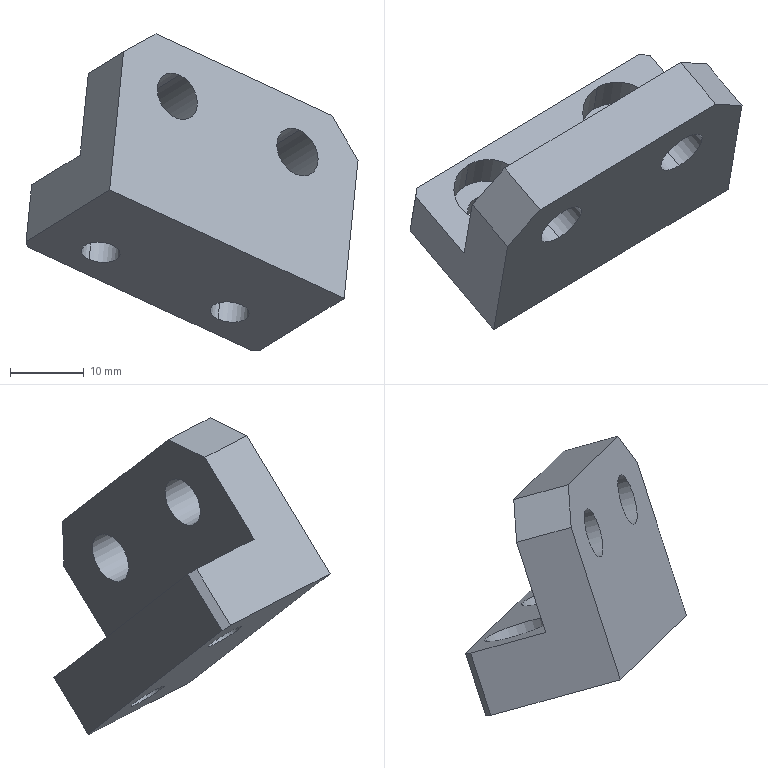Component | SolidWorks | 14AC-24-1-009-2 | 1 solid | 26 faces | box 45.12 x 37.53 x 42.96 mm | volume 11112 mm3 | plane 14 | cylinder 12 | commonest cylinder face diameters 10 x4 5.3 x4 6.8 x2 7 x2
build123d program:
from build123d import *

# Parameters (mm, degrees)
SKETCH1_W                                            = 27
SKETCH1_H                                            = 40
BOSS_EXTRUDE1_DEPTH                                  = 8
M8X1_0_TAPPED_HOLE1_D                                = 7
M8X1_0_TAPPED_HOLE1_DEPTH                            = 19
M8X1_0_TAPPED_HOLE1_TIP                              = 2.103
M8_TAPPED_HOLE1_D                                    = 6.8
M8_TAPPED_HOLE1_DEPTH                                = 19.75
M8_TAPPED_HOLE1_TIP                                  = 2.043
SKETCH6_W                                            = 9
SKETCH6_H                                            = 40
BOSS_EXTRUDE2_DEPTH                                  = 12
HOLE_SIZE_ACCORDING_TO_THE_TYPE_1_OF_HEX_D           = 5.3
HOLE_SIZE_ACCORDING_TO_THE_TYPE_1_OF_HEX_CBORE_D     = 10
HOLE_SIZE_ACCORDING_TO_THE_TYPE_1_OF_HEX_CBORE_DEPTH = 5.7
CHAMFER1_SIZE                                        = 5
CHAMFER2_SIZE                                        = 1


with BuildPart() as part:
    # Sketch1 → Boss-Extrude1 (new body)
    with BuildSketch(Plane.XY):
        Rectangle(SKETCH1_W, SKETCH1_H)
    extrude(amount=BOSS_EXTRUDE1_DEPTH)

    # M8x1.0 Tapped Hole1
    with Locations(Plane(origin=(5.5, 10, 8), x_dir=(1, 0, 0), z_dir=(0, 0, 1))):
        with Locations((0, 0)):
            Hole(M8X1_0_TAPPED_HOLE1_D / 2, depth=M8X1_0_TAPPED_HOLE1_DEPTH)
            with Locations((0, 0, -(M8X1_0_TAPPED_HOLE1_DEPTH + M8X1_0_TAPPED_HOLE1_TIP / 2))):  # 118° drill point
                Cone(0, M8X1_0_TAPPED_HOLE1_D / 2, M8X1_0_TAPPED_HOLE1_TIP, mode=Mode.SUBTRACT)

    # M8 Tapped Hole1
    with Locations(Plane(origin=(5.5, -10.5, 8), x_dir=(1, 0, 0), z_dir=(0, 0, 1))):
        with Locations((0, 0)):
            Hole(M8_TAPPED_HOLE1_D / 2, depth=M8_TAPPED_HOLE1_DEPTH)
            with Locations((0, 0, -(M8_TAPPED_HOLE1_DEPTH + M8_TAPPED_HOLE1_TIP / 2))):  # 118° drill point
                Cone(0, M8_TAPPED_HOLE1_D / 2, M8_TAPPED_HOLE1_TIP, mode=Mode.SUBTRACT)

    # Sketch6 → Boss-Extrude2 (add)
    with BuildSketch(Plane.XY.offset(8)):
        with Locations((-9, 0)):
            Rectangle(SKETCH6_W, SKETCH6_H)
    extrude(amount=BOSS_EXTRUDE2_DEPTH)

    # Hole Size according to the type 1 of hex (through all)
    with Locations(Plane(origin=(-4.5, 11, 14), x_dir=(0, 1, 0), z_dir=(1, 0, 0))):
        with Locations((0, 0), (-22, 0)):
            CounterBoreHole(HOLE_SIZE_ACCORDING_TO_THE_TYPE_1_OF_HEX_D / 2, HOLE_SIZE_ACCORDING_TO_THE_TYPE_1_OF_HEX_CBORE_D / 2, HOLE_SIZE_ACCORDING_TO_THE_TYPE_1_OF_HEX_CBORE_DEPTH)

    # Chamfer1
    chamfer1_edges = [part.edges().sort_by_distance(p)[0] for p in [
        (13.5, -20, 4),
        (13.5, 20, 4),
    ]]
    chamfer(chamfer1_edges, length=CHAMFER1_SIZE)

    # Chamfer2
    chamfer2_edges = [part.edges().sort_by_distance(p)[0] for p in [
        (-9, 20, 20),
        (-9, -20, 20),
    ]]
    chamfer(chamfer2_edges, length=CHAMFER2_SIZE)


solid = part.part

# Placed as in the assembly
solid = solid.moved(Location((533.188, -316.638, -28.905), (-117.442, -36.759, -83.855)))
STEP:
#1=COLOUR_RGB('',0.7922,0.8196,0.9333);
#2=FILL_AREA_STYLE_COLOUR('',#1);
#3=FILL_AREA_STYLE('',(#2));
#4=SURFACE_STYLE_FILL_AREA(#3);
#5=SURFACE_SIDE_STYLE('',(#4));
#6=SURFACE_STYLE_USAGE(.BOTH.,#5);
#7=PRESENTATION_STYLE_ASSIGNMENT((#6));
#8=CARTESIAN_POINT('',(20.855,-11.934,-1.917));
#9=VERTEX_POINT('',#8);
#10=CARTESIAN_POINT('',(21.09,-12.214,-1.771));
#11=VERTEX_POINT('',#10);
#12=CARTESIAN_POINT('',(20.972,-12.074,-1.844));
#13=DIRECTION('',(0.08576,0.5151,0.8529));
#14=DIRECTION('',(0.5985,-0.711,0.3692));
#15=AXIS2_PLACEMENT_3D('',#12,#13,#14);
#16=CIRCLE('',#15,0.1969);
#17=EDGE_CURVE('',#9,#11,#16,.T.);
#18=ORIENTED_EDGE('',*,*,#17,.F.);
#19=CARTESIAN_POINT('',(20.874,-11.818,-1.725));
#20=VERTEX_POINT('',#19);
#21=CARTESIAN_POINT('',(20.874,-11.818,-1.725));
#22=DIRECTION('',(0.08576,0.5151,0.8529));
#23=VECTOR('',#22,39.37);
#24=LINE('',#21,#23);
#25=EDGE_CURVE('',#9,#20,#24,.T.);
#26=ORIENTED_EDGE('',*,*,#25,.T.);
#27=CARTESIAN_POINT('',(21.109,-12.098,-1.58));
#28=VERTEX_POINT('',#27);
#29=CARTESIAN_POINT('',(20.992,-11.958,-1.652));
#30=DIRECTION('',(0.08576,0.5151,0.8529));
#31=DIRECTION('',(0.5985,-0.711,0.3692));
#32=AXIS2_PLACEMENT_3D('',#29,#30,#31);
#33=CIRCLE('',#32,0.1969);
#34=EDGE_CURVE('',#20,#28,#33,.T.);
#35=ORIENTED_EDGE('',*,*,#34,.T.);
#36=CARTESIAN_POINT('',(21.109,-12.098,-1.58));
#37=DIRECTION('',(0.08576,0.5151,0.8529));
#38=VECTOR('',#37,39.37);
#39=LINE('',#36,#38);
#40=EDGE_CURVE('',#11,#28,#39,.T.);
#41=ORIENTED_EDGE('',*,*,#40,.F.);
#42=EDGE_LOOP('',(#18,#26,#35,#41));
#43=FACE_OUTER_BOUND('',#42,.T.);
#44=CARTESIAN_POINT('',(20.992,-11.958,-1.652));
#45=DIRECTION('',(0.08576,0.5151,0.8529));
#46=DIRECTION('',(0.5985,-0.711,0.3692));
#47=AXIS2_PLACEMENT_3D('',#44,#45,#46);
#48=CYLINDRICAL_SURFACE('',#47,0.1969);
#49=ADVANCED_FACE('',(#43),#48,.F.);
#50=CARTESIAN_POINT('',(20.899,-12.066,-1.993));
#51=VERTEX_POINT('',#50);
#52=CARTESIAN_POINT('',(21.024,-12.215,-1.916));
#53=VERTEX_POINT('',#52);
#54=CARTESIAN_POINT('',(20.961,-12.141,-1.955));
#55=DIRECTION('',(0.08576,0.5151,0.8529));
#56=DIRECTION('',(0.5985,-0.711,0.3692));
#57=AXIS2_PLACEMENT_3D('',#54,#55,#56);
#58=CIRCLE('',#57,0.1043);
#59=EDGE_CURVE('',#51,#53,#58,.T.);
#60=ORIENTED_EDGE('',*,*,#59,.F.);
#61=CARTESIAN_POINT('',(20.91,-11.999,-1.882));
#62=VERTEX_POINT('',#61);
#63=CARTESIAN_POINT('',(20.929,-11.884,-1.691));
#64=DIRECTION('',(0.08576,0.5151,0.8529));
#65=VECTOR('',#64,39.37);
#66=LINE('',#63,#65);
#67=EDGE_CURVE('',#51,#62,#66,.T.);
#68=ORIENTED_EDGE('',*,*,#67,.T.);
#69=CARTESIAN_POINT('',(21.035,-12.148,-1.805));
#70=VERTEX_POINT('',#69);
#71=CARTESIAN_POINT('',(20.972,-12.074,-1.844));
#72=DIRECTION('',(0.08576,0.5151,0.8529));
#73=DIRECTION('',(0.5985,-0.711,0.3692));
#74=AXIS2_PLACEMENT_3D('',#71,#72,#73);
#75=CIRCLE('',#74,0.1043);
#76=EDGE_CURVE('',#62,#70,#75,.T.);
#77=ORIENTED_EDGE('',*,*,#76,.T.);
#78=CARTESIAN_POINT('',(21.054,-12.032,-1.614));
#79=DIRECTION('',(0.08576,0.5151,0.8529));
#80=VECTOR('',#79,39.37);
#81=LINE('',#78,#80);
#82=EDGE_CURVE('',#53,#70,#81,.T.);
#83=ORIENTED_EDGE('',*,*,#82,.F.);
#84=EDGE_LOOP('',(#60,#68,#77,#83));
#85=FACE_OUTER_BOUND('',#84,.T.);
#86=CARTESIAN_POINT('',(20.992,-11.958,-1.652));
#87=DIRECTION('',(0.08576,0.5151,0.8529));
#88=DIRECTION('',(0.5985,-0.711,0.3692));
#89=AXIS2_PLACEMENT_3D('',#86,#87,#88);
#90=CYLINDRICAL_SURFACE('',#89,0.1043);
#91=ADVANCED_FACE('',(#85),#90,.F.);
#92=CARTESIAN_POINT('',(20.165,-12.348,-1.597));
#93=VERTEX_POINT('',#92);
#94=CARTESIAN_POINT('',(20.4,-12.628,-1.451));
#95=VERTEX_POINT('',#94);
#96=CARTESIAN_POINT('',(20.282,-12.488,-1.524));
#97=DIRECTION('',(0.08576,0.5151,0.8529));
#98=DIRECTION('',(0.5985,-0.711,0.3692));
#99=AXIS2_PLACEMENT_3D('',#96,#97,#98);
#100=CIRCLE('',#99,0.1969);
#101=EDGE_CURVE('',#93,#95,#100,.T.);
#102=ORIENTED_EDGE('',*,*,#101,.F.);
#103=CARTESIAN_POINT('',(20.184,-12.233,-1.405));
#104=VERTEX_POINT('',#103);
#105=CARTESIAN_POINT('',(20.184,-12.233,-1.405));
#106=DIRECTION('',(0.08576,0.5151,0.8529));
#107=VECTOR('',#106,39.37);
#108=LINE('',#105,#107);
#109=EDGE_CURVE('',#93,#104,#108,.T.);
#110=ORIENTED_EDGE('',*,*,#109,.T.);
#111=CARTESIAN_POINT('',(20.419,-12.513,-1.26));
#112=VERTEX_POINT('',#111);
#113=CARTESIAN_POINT('',(20.302,-12.373,-1.333));
#114=DIRECTION('',(0.08576,0.5151,0.8529));
#115=DIRECTION('',(0.5985,-0.711,0.3692));
#116=AXIS2_PLACEMENT_3D('',#113,#114,#115);
#117=CIRCLE('',#116,0.1969);
#118=EDGE_CURVE('',#104,#112,#117,.T.);
#119=ORIENTED_EDGE('',*,*,#118,.T.);
#120=CARTESIAN_POINT('',(20.419,-12.513,-1.26));
#121=DIRECTION('',(0.08576,0.5151,0.8529));
#122=VECTOR('',#121,39.37);
#123=LINE('',#120,#122);
#124=EDGE_CURVE('',#95,#112,#123,.T.);
#125=ORIENTED_EDGE('',*,*,#124,.F.);
#126=EDGE_LOOP('',(#102,#110,#119,#125));
#127=FACE_OUTER_BOUND('',#126,.T.);
#128=CARTESIAN_POINT('',(20.302,-12.373,-1.333));
#129=DIRECTION('',(0.08576,0.5151,0.8529));
#130=DIRECTION('',(0.5985,-0.711,0.3692));
#131=AXIS2_PLACEMENT_3D('',#128,#129,#130);
#132=CYLINDRICAL_SURFACE('',#131,0.1969);
#133=ADVANCED_FACE('',(#127),#132,.F.);
#134=CARTESIAN_POINT('',(20.209,-12.481,-1.673));
#135=VERTEX_POINT('',#134);
#136=CARTESIAN_POINT('',(20.334,-12.629,-1.596));
#137=VERTEX_POINT('',#136);
#138=CARTESIAN_POINT('',(20.271,-12.555,-1.635));
#139=DIRECTION('',(0.08576,0.5151,0.8529));
#140=DIRECTION('',(0.5985,-0.711,0.3692));
#141=AXIS2_PLACEMENT_3D('',#138,#139,#140);
#142=CIRCLE('',#141,0.1043);
#143=EDGE_CURVE('',#135,#137,#142,.T.);
#144=ORIENTED_EDGE('',*,*,#143,.F.);
#145=CARTESIAN_POINT('',(20.22,-12.414,-1.563));
#146=VERTEX_POINT('',#145);
#147=CARTESIAN_POINT('',(20.239,-12.299,-1.371));
#148=DIRECTION('',(0.08576,0.5151,0.8529));
#149=VECTOR('',#148,39.37);
#150=LINE('',#147,#149);
#151=EDGE_CURVE('',#135,#146,#150,.T.);
#152=ORIENTED_EDGE('',*,*,#151,.T.);
#153=CARTESIAN_POINT('',(20.345,-12.562,-1.486));
#154=VERTEX_POINT('',#153);
#155=CARTESIAN_POINT('',(20.282,-12.488,-1.524));
#156=DIRECTION('',(0.08576,0.5151,0.8529));
#157=DIRECTION('',(0.5985,-0.711,0.3692));
#158=AXIS2_PLACEMENT_3D('',#155,#156,#157);
#159=CIRCLE('',#158,0.1043);
#160=EDGE_CURVE('',#146,#154,#159,.T.);
#161=ORIENTED_EDGE('',*,*,#160,.T.);
#162=CARTESIAN_POINT('',(20.364,-12.447,-1.294));
#163=DIRECTION('',(0.08576,0.5151,0.8529));
#164=VECTOR('',#163,39.37);
#165=LINE('',#162,#164);
#166=EDGE_CURVE('',#137,#154,#165,.T.);
#167=ORIENTED_EDGE('',*,*,#166,.F.);
#168=EDGE_LOOP('',(#144,#152,#161,#167));
#169=FACE_OUTER_BOUND('',#168,.T.);
#170=CARTESIAN_POINT('',(20.302,-12.373,-1.333));
#171=DIRECTION('',(0.08576,0.5151,0.8529));
#172=DIRECTION('',(0.5985,-0.711,0.3692));
#173=AXIS2_PLACEMENT_3D('',#170,#171,#172);
#174=CYLINDRICAL_SURFACE('',#173,0.1043);
#175=ADVANCED_FACE('',(#169),#174,.F.);
#176=CARTESIAN_POINT('',(20.669,-12.621,-0.9148));
#177=VERTEX_POINT('',#176);
#178=CARTESIAN_POINT('',(20.692,-12.483,-0.6865));
#179=VERTEX_POINT('',#178);
#180=CARTESIAN_POINT('',(20.681,-12.552,-0.8007));
#181=DIRECTION('',(-0.5985,0.711,-0.3692));
#182=DIRECTION('',(0.08576,0.5151,0.8529));
#183=AXIS2_PLACEMENT_3D('',#180,#181,#182);
#184=CIRCLE('',#183,0.1339);
#185=EDGE_CURVE('',#177,#179,#184,.T.);
#186=ORIENTED_EDGE('',*,*,#185,.F.);
#187=CARTESIAN_POINT('',(20.481,-12.397,-1.031));
#188=VERTEX_POINT('',#187);
#189=CARTESIAN_POINT('',(20.481,-12.397,-1.031));
#190=DIRECTION('',(-0.5985,0.711,-0.3692));
#191=VECTOR('',#190,39.37);
#192=LINE('',#189,#191);
#193=EDGE_CURVE('',#177,#188,#192,.T.);
#194=ORIENTED_EDGE('',*,*,#193,.T.);
#195=CARTESIAN_POINT('',(20.504,-12.26,-0.8028));
#196=VERTEX_POINT('',#195);
#197=CARTESIAN_POINT('',(20.492,-12.328,-0.917));
#198=DIRECTION('',(-0.5985,0.711,-0.3692));
#199=DIRECTION('',(0.08576,0.5151,0.8529));
#200=AXIS2_PLACEMENT_3D('',#197,#198,#199);
#201=CIRCLE('',#200,0.1339);
#202=EDGE_CURVE('',#188,#196,#201,.T.);
#203=ORIENTED_EDGE('',*,*,#202,.T.);
#204=CARTESIAN_POINT('',(20.504,-12.26,-0.8028));
#205=DIRECTION('',(-0.5985,0.711,-0.3692));
#206=VECTOR('',#205,39.37);
#207=LINE('',#204,#206);
#208=EDGE_CURVE('',#179,#196,#207,.T.);
#209=ORIENTED_EDGE('',*,*,#208,.F.);
#210=EDGE_LOOP('',(#186,#194,#203,#209));
#211=FACE_OUTER_BOUND('',#210,.T.);
#212=CARTESIAN_POINT('',(20.492,-12.328,-0.917));
#213=DIRECTION('',(-0.5985,0.711,-0.3692));
#214=DIRECTION('',(0.08576,0.5151,0.8529));
#215=AXIS2_PLACEMENT_3D('',#212,#213,#214);
#216=CYLINDRICAL_SURFACE('',#215,0.1339);
#217=ADVANCED_FACE('',(#211),#216,.F.);
#218=CARTESIAN_POINT('',(21.312,-12.237,-1.216));
#219=VERTEX_POINT('',#218);
#220=CARTESIAN_POINT('',(21.336,-12.095,-0.9811));
#221=VERTEX_POINT('',#220);
#222=CARTESIAN_POINT('',(21.324,-12.166,-1.099));
#223=DIRECTION('',(-0.5985,0.711,-0.3692));
#224=DIRECTION('',(0.08576,0.5151,0.8529));
#225=AXIS2_PLACEMENT_3D('',#222,#223,#224);
#226=CIRCLE('',#225,0.1378);
#227=EDGE_CURVE('',#219,#221,#226,.T.);
#228=ORIENTED_EDGE('',*,*,#227,.F.);
#229=CARTESIAN_POINT('',(21.124,-12.013,-1.332));
#230=VERTEX_POINT('',#229);
#231=CARTESIAN_POINT('',(21.124,-12.013,-1.332));
#232=DIRECTION('',(-0.5985,0.711,-0.3692));
#233=VECTOR('',#232,39.37);
#234=LINE('',#231,#233);
#235=EDGE_CURVE('',#219,#230,#234,.T.);
#236=ORIENTED_EDGE('',*,*,#235,.T.);
#237=CARTESIAN_POINT('',(21.147,-11.871,-1.097));
#238=VERTEX_POINT('',#237);
#239=CARTESIAN_POINT('',(21.135,-11.942,-1.215));
#240=DIRECTION('',(-0.5985,0.711,-0.3692));
#241=DIRECTION('',(0.08576,0.5151,0.8529));
#242=AXIS2_PLACEMENT_3D('',#239,#240,#241);
#243=CIRCLE('',#242,0.1378);
#244=EDGE_CURVE('',#230,#238,#243,.T.);
#245=ORIENTED_EDGE('',*,*,#244,.T.);
#246=CARTESIAN_POINT('',(21.147,-11.871,-1.097));
#247=DIRECTION('',(-0.5985,0.711,-0.3692));
#248=VECTOR('',#247,39.37);
#249=LINE('',#246,#248);
#250=EDGE_CURVE('',#221,#238,#249,.T.);
#251=ORIENTED_EDGE('',*,*,#250,.F.);
#252=EDGE_LOOP('',(#228,#236,#245,#251));
#253=FACE_OUTER_BOUND('',#252,.T.);
#254=CARTESIAN_POINT('',(21.135,-11.942,-1.215));
#255=DIRECTION('',(-0.5985,0.711,-0.3692));
#256=DIRECTION('',(0.08576,0.5151,0.8529));
#257=AXIS2_PLACEMENT_3D('',#254,#255,#256);
#258=CYLINDRICAL_SURFACE('',#257,0.1378);
#259=ADVANCED_FACE('',(#253),#258,.F.);
#260=CARTESIAN_POINT('',(20.378,-12.251,-0.5829));
#261=VERTEX_POINT('',#260);
#262=CARTESIAN_POINT('',(21.319,-11.686,-1.019));
#263=VERTEX_POINT('',#262);
#264=CARTESIAN_POINT('',(21.476,-11.591,-1.092));
#265=DIRECTION('',(0.7966,0.4787,-0.3692));
#266=VECTOR('',#265,39.37);
#267=LINE('',#264,#266);
#268=EDGE_CURVE('',#261,#263,#267,.T.);
#269=ORIENTED_EDGE('',*,*,#268,.F.);
#270=CARTESIAN_POINT('',(20.567,-12.475,-0.4666));
#271=VERTEX_POINT('',#270);
#272=CARTESIAN_POINT('',(20.378,-12.251,-0.5829));
#273=DIRECTION('',(0.5985,-0.711,0.3692));
#274=VECTOR('',#273,39.37);
#275=LINE('',#272,#274);
#276=EDGE_CURVE('',#261,#271,#275,.T.);
#277=ORIENTED_EDGE('',*,*,#276,.T.);
#278=CARTESIAN_POINT('',(21.508,-11.91,-0.9027));
#279=VERTEX_POINT('',#278);
#280=CARTESIAN_POINT('',(21.664,-11.815,-0.9754));
#281=DIRECTION('',(0.7966,0.4787,-0.3692));
#282=VECTOR('',#281,39.37);
#283=LINE('',#280,#282);
#284=EDGE_CURVE('',#271,#279,#283,.T.);
#285=ORIENTED_EDGE('',*,*,#284,.T.);
#286=CARTESIAN_POINT('',(21.319,-11.686,-1.019));
#287=DIRECTION('',(-0.5985,0.711,-0.3692));
#288=VECTOR('',#287,39.37);
#289=LINE('',#286,#288);
#290=EDGE_CURVE('',#279,#263,#289,.T.);
#291=ORIENTED_EDGE('',*,*,#290,.T.);
#292=EDGE_LOOP('',(#269,#277,#285,#291));
#293=FACE_OUTER_BOUND('',#292,.T.);
#294=CARTESIAN_POINT('',(21.476,-11.591,-1.092));
#295=DIRECTION('',(-0.08576,-0.5151,-0.8529));
#296=DIRECTION('',(-0.7966,-0.4787,0.3692));
#297=AXIS2_PLACEMENT_3D('',#294,#295,#296);
#298=PLANE('',#297);
#299=ADVANCED_FACE('',(#293),#298,.F.);
#300=CARTESIAN_POINT('',(21.126,-11.831,-2.158));
#301=VERTEX_POINT('',#300);
#302=CARTESIAN_POINT('',(21.573,-12.363,-1.882));
#303=VERTEX_POINT('',#302);
#304=CARTESIAN_POINT('',(21.385,-12.139,-1.998));
#305=DIRECTION('',(0.5985,-0.711,0.3692));
#306=VECTOR('',#305,39.37);
#307=LINE('',#304,#306);
#308=EDGE_CURVE('',#301,#303,#307,.T.);
#309=ORIENTED_EDGE('',*,*,#308,.F.);
#310=CARTESIAN_POINT('',(21.156,-11.648,-1.856));
#311=VERTEX_POINT('',#310);
#312=CARTESIAN_POINT('',(21.156,-11.648,-1.856));
#313=DIRECTION('',(0.08576,0.5151,0.8529));
#314=VECTOR('',#313,39.37);
#315=LINE('',#312,#314);
#316=EDGE_CURVE('',#301,#311,#315,.T.);
#317=ORIENTED_EDGE('',*,*,#316,.T.);
#318=CARTESIAN_POINT('',(21.415,-11.956,-1.696));
#319=VERTEX_POINT('',#318);
#320=CARTESIAN_POINT('',(21.132,-11.621,-1.871));
#321=DIRECTION('',(0.5985,-0.711,0.3692));
#322=VECTOR('',#321,39.37);
#323=LINE('',#320,#322);
#324=EDGE_CURVE('',#311,#319,#323,.T.);
#325=ORIENTED_EDGE('',*,*,#324,.T.);
#326=CARTESIAN_POINT('',(21.459,-11.693,-1.26));
#327=VERTEX_POINT('',#326);
#328=CARTESIAN_POINT('',(21.385,-12.139,-1.998));
#329=DIRECTION('',(-0.08576,-0.5151,-0.8529));
#330=VECTOR('',#329,39.37);
#331=LINE('',#328,#330);
#332=EDGE_CURVE('',#327,#319,#331,.T.);
#333=ORIENTED_EDGE('',*,*,#332,.F.);
#334=CARTESIAN_POINT('',(21.648,-11.917,-1.143));
#335=VERTEX_POINT('',#334);
#336=CARTESIAN_POINT('',(21.459,-11.693,-1.26));
#337=DIRECTION('',(0.5985,-0.711,0.3692));
#338=VECTOR('',#337,39.37);
#339=LINE('',#336,#338);
#340=EDGE_CURVE('',#327,#335,#339,.T.);
#341=ORIENTED_EDGE('',*,*,#340,.T.);
#342=CARTESIAN_POINT('',(21.573,-12.363,-1.882));
#343=DIRECTION('',(-0.08576,-0.5151,-0.8529));
#344=VECTOR('',#343,39.37);
#345=LINE('',#342,#344);
#346=EDGE_CURVE('',#335,#303,#345,.T.);
#347=ORIENTED_EDGE('',*,*,#346,.T.);
#348=EDGE_LOOP('',(#309,#317,#325,#333,#341,#347));
#349=FACE_OUTER_BOUND('',#348,.T.);
#350=CARTESIAN_POINT('',(21.385,-12.139,-1.998));
#351=DIRECTION('',(-0.7966,-0.4787,0.3692));
#352=DIRECTION('',(0.5985,-0.711,0.3692));
#353=AXIS2_PLACEMENT_3D('',#350,#351,#352);
#354=PLANE('',#353);
#355=ADVANCED_FACE('',(#349),#354,.F.);
#356=CARTESIAN_POINT('',(20.961,-12.141,-1.955));
#357=DIRECTION('',(0.08576,0.5151,0.8529));
#358=DIRECTION('',(0.5985,-0.711,0.3692));
#359=AXIS2_PLACEMENT_3D('',#356,#357,#358);
#360=CIRCLE('',#359,0.1043);
#361=EDGE_CURVE('',#53,#51,#360,.T.);
#362=ORIENTED_EDGE('',*,*,#361,.T.);
#363=ORIENTED_EDGE('',*,*,#59,.T.);
#364=EDGE_LOOP('',(#362,#363));
#365=FACE_BOUND('',#364,.T.);
#366=CARTESIAN_POINT('',(20.271,-12.555,-1.635));
#367=DIRECTION('',(0.08576,0.5151,0.8529));
#368=DIRECTION('',(0.5985,-0.711,0.3692));
#369=AXIS2_PLACEMENT_3D('',#366,#367,#368);
#370=CIRCLE('',#369,0.1043);
#371=EDGE_CURVE('',#137,#135,#370,.T.);
#372=ORIENTED_EDGE('',*,*,#371,.T.);
#373=ORIENTED_EDGE('',*,*,#143,.T.);
#374=EDGE_LOOP('',(#372,#373));
#375=FACE_BOUND('',#374,.T.);
#376=CARTESIAN_POINT('',(21.071,-11.822,-2.158));
#377=VERTEX_POINT('',#376);
#378=CARTESIAN_POINT('',(19.879,-12.538,-1.606));
#379=VERTEX_POINT('',#378);
#380=CARTESIAN_POINT('',(21.102,-11.803,-2.173));
#381=DIRECTION('',(-0.7966,-0.4787,0.3692));
#382=VECTOR('',#381,39.37);
#383=LINE('',#380,#382);
#384=EDGE_CURVE('',#377,#379,#383,.T.);
#385=ORIENTED_EDGE('',*,*,#384,.F.);
#386=CARTESIAN_POINT('',(21.071,-11.822,-2.158));
#387=DIRECTION('',(0.9864,-0.1642,0.));
#388=VECTOR('',#387,39.37);
#389=LINE('',#386,#388);
#390=EDGE_CURVE('',#377,#301,#389,.T.);
#391=ORIENTED_EDGE('',*,*,#390,.T.);
#392=ORIENTED_EDGE('',*,*,#308,.T.);
#393=CARTESIAN_POINT('',(20.319,-13.117,-1.301));
#394=VERTEX_POINT('',#393);
#395=CARTESIAN_POINT('',(21.573,-12.363,-1.882));
#396=DIRECTION('',(-0.7966,-0.4787,0.3692));
#397=VECTOR('',#396,39.37);
#398=LINE('',#395,#397);
#399=EDGE_CURVE('',#303,#394,#398,.T.);
#400=ORIENTED_EDGE('',*,*,#399,.T.);
#401=CARTESIAN_POINT('',(19.871,-12.585,-1.577));
#402=VERTEX_POINT('',#401);
#403=CARTESIAN_POINT('',(20.13,-12.893,-1.417));
#404=DIRECTION('',(0.5985,-0.711,0.3692));
#405=VECTOR('',#404,39.37);
#406=LINE('',#403,#405);
#407=EDGE_CURVE('',#402,#394,#406,.T.);
#408=ORIENTED_EDGE('',*,*,#407,.F.);
#409=CARTESIAN_POINT('',(19.879,-12.538,-1.606));
#410=DIRECTION('',(0.1401,0.8413,-0.5222));
#411=VECTOR('',#410,39.37);
#412=LINE('',#409,#411);
#413=EDGE_CURVE('',#402,#379,#412,.T.);
#414=ORIENTED_EDGE('',*,*,#413,.T.);
#415=EDGE_LOOP('',(#385,#391,#392,#400,#408,#414));
#416=FACE_OUTER_BOUND('',#415,.T.);
#417=CARTESIAN_POINT('',(21.385,-12.139,-1.998));
#418=DIRECTION('',(0.08576,0.5151,0.8529));
#419=DIRECTION('',(0.7966,0.4787,-0.3692));
#420=AXIS2_PLACEMENT_3D('',#417,#418,#419);
#421=PLANE('',#420);
#422=ADVANCED_FACE('',(#365,#375,#416),#421,.F.);
#423=CARTESIAN_POINT('',(19.902,-12.402,-1.275));
#424=VERTEX_POINT('',#423);
#425=CARTESIAN_POINT('',(20.161,-12.71,-1.115));
#426=VERTEX_POINT('',#425);
#427=CARTESIAN_POINT('',(19.878,-12.374,-1.289));
#428=DIRECTION('',(0.5985,-0.711,0.3692));
#429=VECTOR('',#428,39.37);
#430=LINE('',#427,#429);
#431=EDGE_CURVE('',#424,#426,#430,.T.);
#432=ORIENTED_EDGE('',*,*,#431,.F.);
#433=CARTESIAN_POINT('',(19.871,-12.585,-1.577));
#434=DIRECTION('',(-0.08576,-0.5151,-0.8529));
#435=VECTOR('',#434,39.37);
#436=LINE('',#433,#435);
#437=EDGE_CURVE('',#424,#402,#436,.T.);
#438=ORIENTED_EDGE('',*,*,#437,.T.);
#439=ORIENTED_EDGE('',*,*,#407,.T.);
#440=CARTESIAN_POINT('',(20.393,-12.671,-0.5618));
#441=VERTEX_POINT('',#440);
#442=CARTESIAN_POINT('',(20.319,-13.117,-1.301));
#443=DIRECTION('',(0.08576,0.5151,0.8529));
#444=VECTOR('',#443,39.37);
#445=LINE('',#442,#444);
#446=EDGE_CURVE('',#394,#441,#445,.T.);
#447=ORIENTED_EDGE('',*,*,#446,.T.);
#448=CARTESIAN_POINT('',(20.205,-12.447,-0.6781));
#449=VERTEX_POINT('',#448);
#450=CARTESIAN_POINT('',(20.205,-12.447,-0.6781));
#451=DIRECTION('',(-0.5985,0.711,-0.3692));
#452=VECTOR('',#451,39.37);
#453=LINE('',#450,#452);
#454=EDGE_CURVE('',#441,#449,#453,.T.);
#455=ORIENTED_EDGE('',*,*,#454,.T.);
#456=CARTESIAN_POINT('',(20.13,-12.893,-1.417));
#457=DIRECTION('',(0.08576,0.5151,0.8529));
#458=VECTOR('',#457,39.37);
#459=LINE('',#456,#458);
#460=EDGE_CURVE('',#426,#449,#459,.T.);
#461=ORIENTED_EDGE('',*,*,#460,.F.);
#462=EDGE_LOOP('',(#432,#438,#439,#447,#455,#461));
#463=FACE_OUTER_BOUND('',#462,.T.);
#464=CARTESIAN_POINT('',(20.13,-12.893,-1.417));
#465=DIRECTION('',(0.7966,0.4787,-0.3692));
#466=DIRECTION('',(-0.5985,0.711,-0.3692));
#467=AXIS2_PLACEMENT_3D('',#464,#465,#466);
#468=PLANE('',#467);
#469=ADVANCED_FACE('',(#463),#468,.F.);
#470=ORIENTED_EDGE('',*,*,#460,.T.);
#471=CARTESIAN_POINT('',(20.404,-12.222,-0.5687));
#472=DIRECTION('',(0.6239,0.7027,0.342));
#473=VECTOR('',#472,39.37);
#474=LINE('',#471,#473);
#475=EDGE_CURVE('',#449,#261,#474,.T.);
#476=ORIENTED_EDGE('',*,*,#475,.T.);
#477=ORIENTED_EDGE('',*,*,#268,.T.);
#478=CARTESIAN_POINT('',(21.298,-11.685,-0.9829));
#479=DIRECTION('',(0.5026,-0.0257,-0.8641));
#480=VECTOR('',#479,39.37);
#481=LINE('',#478,#480);
#482=EDGE_CURVE('',#263,#327,#481,.T.);
#483=ORIENTED_EDGE('',*,*,#482,.T.);
#484=ORIENTED_EDGE('',*,*,#332,.T.);
#485=CARTESIAN_POINT('',(21.415,-11.956,-1.696));
#486=DIRECTION('',(0.7966,0.4787,-0.3692));
#487=VECTOR('',#486,39.37);
#488=LINE('',#485,#487);
#489=EDGE_CURVE('',#426,#319,#488,.T.);
#490=ORIENTED_EDGE('',*,*,#489,.F.);
#491=EDGE_LOOP('',(#470,#476,#477,#483,#484,#490));
#492=FACE_OUTER_BOUND('',#491,.T.);
#493=CARTESIAN_POINT('',(20.492,-12.328,-0.917));
#494=DIRECTION('',(-0.5985,0.711,-0.3692));
#495=DIRECTION('',(0.08576,0.5151,0.8529));
#496=AXIS2_PLACEMENT_3D('',#493,#494,#495);
#497=CIRCLE('',#496,0.1339);
#498=EDGE_CURVE('',#196,#188,#497,.T.);
#499=ORIENTED_EDGE('',*,*,#498,.F.);
#500=ORIENTED_EDGE('',*,*,#202,.F.);
#501=EDGE_LOOP('',(#499,#500));
#502=FACE_BOUND('',#501,.T.);
#503=CARTESIAN_POINT('',(21.135,-11.942,-1.215));
#504=DIRECTION('',(-0.5985,0.711,-0.3692));
#505=DIRECTION('',(0.08576,0.5151,0.8529));
#506=AXIS2_PLACEMENT_3D('',#503,#504,#505);
#507=CIRCLE('',#506,0.1378);
#508=EDGE_CURVE('',#238,#230,#507,.T.);
#509=ORIENTED_EDGE('',*,*,#508,.F.);
#510=ORIENTED_EDGE('',*,*,#244,.F.);
#511=EDGE_LOOP('',(#509,#510));
#512=FACE_BOUND('',#511,.T.);
#513=CARTESIAN_POINT('',(20.803,-12.242,-1.254));
#514=DIRECTION('',(-0.5985,0.711,-0.3692));
#515=DIRECTION('',(0.08576,0.5151,0.8529));
#516=AXIS2_PLACEMENT_3D('',#513,#514,#515);
#517=PLANE('',#516);
#518=ADVANCED_FACE('',(#492,#502,#512),#517,.T.);
#519=CARTESIAN_POINT('',(20.681,-12.552,-0.8007));
#520=DIRECTION('',(-0.5985,0.711,-0.3692));
#521=DIRECTION('',(0.08576,0.5151,0.8529));
#522=AXIS2_PLACEMENT_3D('',#519,#520,#521);
#523=CIRCLE('',#522,0.1339);
#524=EDGE_CURVE('',#179,#177,#523,.T.);
#525=ORIENTED_EDGE('',*,*,#524,.T.);
#526=ORIENTED_EDGE('',*,*,#185,.T.);
#527=EDGE_LOOP('',(#525,#526));
#528=FACE_BOUND('',#527,.T.);
#529=CARTESIAN_POINT('',(21.324,-12.166,-1.099));
#530=DIRECTION('',(-0.5985,0.711,-0.3692));
#531=DIRECTION('',(0.08576,0.5151,0.8529));
#532=AXIS2_PLACEMENT_3D('',#529,#530,#531);
#533=CIRCLE('',#532,0.1378);
#534=EDGE_CURVE('',#221,#219,#533,.T.);
#535=ORIENTED_EDGE('',*,*,#534,.T.);
#536=ORIENTED_EDGE('',*,*,#227,.T.);
#537=EDGE_LOOP('',(#535,#536));
#538=FACE_BOUND('',#537,.T.);
#539=ORIENTED_EDGE('',*,*,#284,.F.);
#540=CARTESIAN_POINT('',(20.567,-12.475,-0.4666));
#541=DIRECTION('',(-0.6239,-0.7027,-0.342));
#542=VECTOR('',#541,39.37);
#543=LINE('',#540,#542);
#544=EDGE_CURVE('',#271,#441,#543,.T.);
#545=ORIENTED_EDGE('',*,*,#544,.T.);
#546=ORIENTED_EDGE('',*,*,#446,.F.);
#547=ORIENTED_EDGE('',*,*,#399,.F.);
#548=ORIENTED_EDGE('',*,*,#346,.F.);
#549=CARTESIAN_POINT('',(21.648,-11.917,-1.143));
#550=DIRECTION('',(-0.5026,0.0257,0.8641));
#551=VECTOR('',#550,39.37);
#552=LINE('',#549,#551);
#553=EDGE_CURVE('',#335,#279,#552,.T.);
#554=ORIENTED_EDGE('',*,*,#553,.T.);
#555=EDGE_LOOP('',(#539,#545,#546,#547,#548,#554));
#556=FACE_OUTER_BOUND('',#555,.T.);
#557=CARTESIAN_POINT('',(20.992,-12.466,-1.138));
#558=DIRECTION('',(-0.5985,0.711,-0.3692));
#559=DIRECTION('',(0.08576,0.5151,0.8529));
#560=AXIS2_PLACEMENT_3D('',#557,#558,#559);
#561=PLANE('',#560);
#562=ADVANCED_FACE('',(#528,#538,#556),#561,.F.);
#563=ORIENTED_EDGE('',*,*,#235,.F.);
#564=ORIENTED_EDGE('',*,*,#534,.F.);
#565=ORIENTED_EDGE('',*,*,#250,.T.);
#566=ORIENTED_EDGE('',*,*,#508,.T.);
#567=EDGE_LOOP('',(#563,#564,#565,#566));
#568=FACE_OUTER_BOUND('',#567,.T.);
#569=CARTESIAN_POINT('',(21.135,-11.942,-1.215));
#570=DIRECTION('',(-0.5985,0.711,-0.3692));
#571=DIRECTION('',(0.08576,0.5151,0.8529));
#572=AXIS2_PLACEMENT_3D('',#569,#570,#571);
#573=CYLINDRICAL_SURFACE('',#572,0.1378);
#574=ADVANCED_FACE('',(#568),#573,.F.);
#575=ORIENTED_EDGE('',*,*,#193,.F.);
#576=ORIENTED_EDGE('',*,*,#524,.F.);
#577=ORIENTED_EDGE('',*,*,#208,.T.);
#578=ORIENTED_EDGE('',*,*,#498,.T.);
#579=EDGE_LOOP('',(#575,#576,#577,#578));
#580=FACE_OUTER_BOUND('',#579,.T.);
#581=CARTESIAN_POINT('',(20.492,-12.328,-0.917));
#582=DIRECTION('',(-0.5985,0.711,-0.3692));
#583=DIRECTION('',(0.08576,0.5151,0.8529));
#584=AXIS2_PLACEMENT_3D('',#581,#582,#583);
#585=CYLINDRICAL_SURFACE('',#584,0.1339);
#586=ADVANCED_FACE('',(#580),#585,.F.);
#587=CARTESIAN_POINT('',(20.992,-11.958,-1.652));
#588=DIRECTION('',(0.08576,0.5151,0.8529));
#589=DIRECTION('',(0.5985,-0.711,0.3692));
#590=AXIS2_PLACEMENT_3D('',#587,#588,#589);
#591=CIRCLE('',#590,0.1969);
#592=EDGE_CURVE('',#28,#20,#591,.T.);
#593=ORIENTED_EDGE('',*,*,#592,.F.);
#594=ORIENTED_EDGE('',*,*,#34,.F.);
#595=EDGE_LOOP('',(#593,#594));
#596=FACE_BOUND('',#595,.T.);
#597=CARTESIAN_POINT('',(20.302,-12.373,-1.333));
#598=DIRECTION('',(0.08576,0.5151,0.8529));
#599=DIRECTION('',(0.5985,-0.711,0.3692));
#600=AXIS2_PLACEMENT_3D('',#597,#598,#599);
#601=CIRCLE('',#600,0.1969);
#602=EDGE_CURVE('',#112,#104,#601,.T.);
#603=ORIENTED_EDGE('',*,*,#602,.F.);
#604=ORIENTED_EDGE('',*,*,#118,.F.);
#605=EDGE_LOOP('',(#603,#604));
#606=FACE_BOUND('',#605,.T.);
#607=ORIENTED_EDGE('',*,*,#324,.F.);
#608=CARTESIAN_POINT('',(21.101,-11.639,-1.856));
#609=VERTEX_POINT('',#608);
#610=CARTESIAN_POINT('',(21.101,-11.639,-1.856));
#611=DIRECTION('',(-0.9864,0.1642,-0.));
#612=VECTOR('',#611,39.37);
#613=LINE('',#610,#612);
#614=EDGE_CURVE('',#311,#609,#613,.T.);
#615=ORIENTED_EDGE('',*,*,#614,.T.);
#616=CARTESIAN_POINT('',(19.909,-12.356,-1.304));
#617=VERTEX_POINT('',#616);
#618=CARTESIAN_POINT('',(21.132,-11.621,-1.871));
#619=DIRECTION('',(0.7966,0.4787,-0.3692));
#620=VECTOR('',#619,39.37);
#621=LINE('',#618,#620);
#622=EDGE_CURVE('',#617,#609,#621,.T.);
#623=ORIENTED_EDGE('',*,*,#622,.F.);
#624=CARTESIAN_POINT('',(19.909,-12.356,-1.304));
#625=DIRECTION('',(-0.1401,-0.8413,0.5222));
#626=VECTOR('',#625,39.37);
#627=LINE('',#624,#626);
#628=EDGE_CURVE('',#617,#424,#627,.T.);
#629=ORIENTED_EDGE('',*,*,#628,.T.);
#630=ORIENTED_EDGE('',*,*,#431,.T.);
#631=ORIENTED_EDGE('',*,*,#489,.T.);
#632=EDGE_LOOP('',(#607,#615,#623,#629,#630,#631));
#633=FACE_OUTER_BOUND('',#632,.T.);
#634=CARTESIAN_POINT('',(21.132,-11.621,-1.871));
#635=DIRECTION('',(-0.08576,-0.5151,-0.8529));
#636=DIRECTION('',(-0.7966,-0.4787,0.3692));
#637=AXIS2_PLACEMENT_3D('',#634,#635,#636);
#638=PLANE('',#637);
#639=ADVANCED_FACE('',(#596,#606,#633),#638,.F.);
#640=ORIENTED_EDGE('',*,*,#622,.T.);
#641=CARTESIAN_POINT('',(21.071,-11.822,-2.158));
#642=DIRECTION('',(-0.08576,-0.5151,-0.8529));
#643=VECTOR('',#642,39.37);
#644=LINE('',#641,#643);
#645=EDGE_CURVE('',#609,#377,#644,.T.);
#646=ORIENTED_EDGE('',*,*,#645,.T.);
#647=ORIENTED_EDGE('',*,*,#384,.T.);
#648=CARTESIAN_POINT('',(19.909,-12.356,-1.304));
#649=DIRECTION('',(0.08576,0.5151,0.8529));
#650=VECTOR('',#649,39.37);
#651=LINE('',#648,#650);
#652=EDGE_CURVE('',#379,#617,#651,.T.);
#653=ORIENTED_EDGE('',*,*,#652,.T.);
#654=EDGE_LOOP('',(#640,#646,#647,#653));
#655=FACE_OUTER_BOUND('',#654,.T.);
#656=CARTESIAN_POINT('',(20.52,-11.906,-1.429));
#657=DIRECTION('',(-0.5985,0.711,-0.3692));
#658=DIRECTION('',(0.08576,0.5151,0.8529));
#659=AXIS2_PLACEMENT_3D('',#656,#657,#658);
#660=PLANE('',#659);
#661=ADVANCED_FACE('',(#655),#660,.T.);
#662=ORIENTED_EDGE('',*,*,#151,.F.);
#663=ORIENTED_EDGE('',*,*,#371,.F.);
#664=ORIENTED_EDGE('',*,*,#166,.T.);
#665=CARTESIAN_POINT('',(20.282,-12.488,-1.524));
#666=DIRECTION('',(0.08576,0.5151,0.8529));
#667=DIRECTION('',(0.5985,-0.711,0.3692));
#668=AXIS2_PLACEMENT_3D('',#665,#666,#667);
#669=CIRCLE('',#668,0.1043);
#670=EDGE_CURVE('',#154,#146,#669,.T.);
#671=ORIENTED_EDGE('',*,*,#670,.T.);
#672=EDGE_LOOP('',(#662,#663,#664,#671));
#673=FACE_OUTER_BOUND('',#672,.T.);
#674=CARTESIAN_POINT('',(20.302,-12.373,-1.333));
#675=DIRECTION('',(0.08576,0.5151,0.8529));
#676=DIRECTION('',(0.5985,-0.711,0.3692));
#677=AXIS2_PLACEMENT_3D('',#674,#675,#676);
#678=CYLINDRICAL_SURFACE('',#677,0.1043);
#679=ADVANCED_FACE('',(#673),#678,.F.);
#680=ORIENTED_EDGE('',*,*,#670,.F.);
#681=ORIENTED_EDGE('',*,*,#160,.F.);
#682=EDGE_LOOP('',(#680,#681));
#683=FACE_BOUND('',#682,.T.);
#684=CARTESIAN_POINT('',(20.282,-12.488,-1.524));
#685=DIRECTION('',(0.08576,0.5151,0.8529));
#686=DIRECTION('',(0.5985,-0.711,0.3692));
#687=AXIS2_PLACEMENT_3D('',#684,#685,#686);
#688=CIRCLE('',#687,0.1969);
#689=EDGE_CURVE('',#95,#93,#688,.T.);
#690=ORIENTED_EDGE('',*,*,#689,.T.);
#691=ORIENTED_EDGE('',*,*,#101,.T.);
#692=EDGE_LOOP('',(#690,#691));
#693=FACE_OUTER_BOUND('',#692,.T.);
#694=CARTESIAN_POINT('',(20.365,-12.438,-1.563));
#695=DIRECTION('',(-0.08576,-0.5151,-0.8529));
#696=DIRECTION('',(-0.5985,0.711,-0.3692));
#697=AXIS2_PLACEMENT_3D('',#694,#695,#696);
#698=PLANE('',#697);
#699=ADVANCED_FACE('',(#683,#693),#698,.F.);
#700=ORIENTED_EDGE('',*,*,#109,.F.);
#701=ORIENTED_EDGE('',*,*,#689,.F.);
#702=ORIENTED_EDGE('',*,*,#124,.T.);
#703=ORIENTED_EDGE('',*,*,#602,.T.);
#704=EDGE_LOOP('',(#700,#701,#702,#703));
#705=FACE_OUTER_BOUND('',#704,.T.);
#706=CARTESIAN_POINT('',(20.302,-12.373,-1.333));
#707=DIRECTION('',(0.08576,0.5151,0.8529));
#708=DIRECTION('',(0.5985,-0.711,0.3692));
#709=AXIS2_PLACEMENT_3D('',#706,#707,#708);
#710=CYLINDRICAL_SURFACE('',#709,0.1969);
#711=ADVANCED_FACE('',(#705),#710,.F.);
#712=ORIENTED_EDGE('',*,*,#67,.F.);
#713=ORIENTED_EDGE('',*,*,#361,.F.);
#714=ORIENTED_EDGE('',*,*,#82,.T.);
#715=CARTESIAN_POINT('',(20.972,-12.074,-1.844));
#716=DIRECTION('',(0.08576,0.5151,0.8529));
#717=DIRECTION('',(0.5985,-0.711,0.3692));
#718=AXIS2_PLACEMENT_3D('',#715,#716,#717);
#719=CIRCLE('',#718,0.1043);
#720=EDGE_CURVE('',#70,#62,#719,.T.);
#721=ORIENTED_EDGE('',*,*,#720,.T.);
#722=EDGE_LOOP('',(#712,#713,#714,#721));
#723=FACE_OUTER_BOUND('',#722,.T.);
#724=CARTESIAN_POINT('',(20.992,-11.958,-1.652));
#725=DIRECTION('',(0.08576,0.5151,0.8529));
#726=DIRECTION('',(0.5985,-0.711,0.3692));
#727=AXIS2_PLACEMENT_3D('',#724,#725,#726);
#728=CYLINDRICAL_SURFACE('',#727,0.1043);
#729=ADVANCED_FACE('',(#723),#728,.F.);
#730=ORIENTED_EDGE('',*,*,#720,.F.);
#731=ORIENTED_EDGE('',*,*,#76,.F.);
#732=EDGE_LOOP('',(#730,#731));
#733=FACE_BOUND('',#732,.T.);
#734=CARTESIAN_POINT('',(20.972,-12.074,-1.844));
#735=DIRECTION('',(0.08576,0.5151,0.8529));
#736=DIRECTION('',(0.5985,-0.711,0.3692));
#737=AXIS2_PLACEMENT_3D('',#734,#735,#736);
#738=CIRCLE('',#737,0.1969);
#739=EDGE_CURVE('',#11,#9,#738,.T.);
#740=ORIENTED_EDGE('',*,*,#739,.T.);
#741=ORIENTED_EDGE('',*,*,#17,.T.);
#742=EDGE_LOOP('',(#740,#741));
#743=FACE_OUTER_BOUND('',#742,.T.);
#744=CARTESIAN_POINT('',(21.055,-12.024,-1.882));
#745=DIRECTION('',(-0.08576,-0.5151,-0.8529));
#746=DIRECTION('',(-0.5985,0.711,-0.3692));
#747=AXIS2_PLACEMENT_3D('',#744,#745,#746);
#748=PLANE('',#747);
#749=ADVANCED_FACE('',(#733,#743),#748,.F.);
#750=ORIENTED_EDGE('',*,*,#25,.F.);
#751=ORIENTED_EDGE('',*,*,#739,.F.);
#752=ORIENTED_EDGE('',*,*,#40,.T.);
#753=ORIENTED_EDGE('',*,*,#592,.T.);
#754=EDGE_LOOP('',(#750,#751,#752,#753));
#755=FACE_OUTER_BOUND('',#754,.T.);
#756=CARTESIAN_POINT('',(20.992,-11.958,-1.652));
#757=DIRECTION('',(0.08576,0.5151,0.8529));
#758=DIRECTION('',(0.5985,-0.711,0.3692));
#759=AXIS2_PLACEMENT_3D('',#756,#757,#758);
#760=CYLINDRICAL_SURFACE('',#759,0.1969);
#761=ADVANCED_FACE('',(#755),#760,.F.);
#762=ORIENTED_EDGE('',*,*,#475,.F.);
#763=ORIENTED_EDGE('',*,*,#454,.F.);
#764=ORIENTED_EDGE('',*,*,#544,.F.);
#765=ORIENTED_EDGE('',*,*,#276,.F.);
#766=EDGE_LOOP('',(#762,#763,#764,#765));
#767=FACE_OUTER_BOUND('',#766,.T.);
#768=CARTESIAN_POINT('',(20.378,-12.251,-0.5829));
#769=DIRECTION('',(0.5026,-0.0257,-0.8641));
#770=DIRECTION('',(0.5985,-0.711,0.3692));
#771=AXIS2_PLACEMENT_3D('',#768,#769,#770);
#772=PLANE('',#771);
#773=ADVANCED_FACE('',(#767),#772,.F.);
#774=ORIENTED_EDGE('',*,*,#482,.F.);
#775=ORIENTED_EDGE('',*,*,#290,.F.);
#776=ORIENTED_EDGE('',*,*,#553,.F.);
#777=ORIENTED_EDGE('',*,*,#340,.F.);
#778=EDGE_LOOP('',(#774,#775,#776,#777));
#779=FACE_OUTER_BOUND('',#778,.T.);
#780=CARTESIAN_POINT('',(21.459,-11.693,-1.26));
#781=DIRECTION('',(-0.6239,-0.7027,-0.342));
#782=DIRECTION('',(0.5985,-0.711,0.3692));
#783=AXIS2_PLACEMENT_3D('',#780,#781,#782);
#784=PLANE('',#783);
#785=ADVANCED_FACE('',(#779),#784,.F.);
#786=ORIENTED_EDGE('',*,*,#614,.F.);
#787=ORIENTED_EDGE('',*,*,#316,.F.);
#788=ORIENTED_EDGE('',*,*,#390,.F.);
#789=ORIENTED_EDGE('',*,*,#645,.F.);
#790=EDGE_LOOP('',(#786,#787,#788,#789));
#791=FACE_OUTER_BOUND('',#790,.T.);
#792=CARTESIAN_POINT('',(21.116,-11.548,-1.705));
#793=DIRECTION('',(0.1401,0.8413,-0.5222));
#794=DIRECTION('',(0.08576,0.5151,0.8529));
#795=AXIS2_PLACEMENT_3D('',#792,#793,#794);
#796=PLANE('',#795);
#797=ADVANCED_FACE('',(#791),#796,.T.);
#798=ORIENTED_EDGE('',*,*,#413,.F.);
#799=ORIENTED_EDGE('',*,*,#437,.F.);
#800=ORIENTED_EDGE('',*,*,#628,.F.);
#801=ORIENTED_EDGE('',*,*,#652,.F.);
#802=EDGE_LOOP('',(#798,#799,#800,#801));
#803=FACE_OUTER_BOUND('',#802,.T.);
#804=CARTESIAN_POINT('',(19.925,-12.264,-1.153));
#805=DIRECTION('',(-0.9864,0.1642,0.));
#806=DIRECTION('',(-0.08576,-0.5151,-0.8529));
#807=AXIS2_PLACEMENT_3D('',#804,#805,#806);
#808=PLANE('',#807);
#809=ADVANCED_FACE('',(#803),#808,.T.);
#810=CLOSED_SHELL('',(#49,#91,#133,#175,#217,#259,#299,#355,#422,#469,#518,#562,#574,#586,#639,#661,#679,#699,#711,#729,#749,#761,#773,#785,#797,#809));
#811=MANIFOLD_SOLID_BREP('',#810);
#812=STYLED_ITEM('',(#7),#811);
#813=PRESENTATION_LAYER_ASSIGNMENT('','',(#812));
#814=CARTESIAN_POINT('',(0.,0.,0.));
#815=DIRECTION('',(0.,0.,1.));
#816=DIRECTION('',(1.,0.,0.));
#817=AXIS2_PLACEMENT_3D('',#814,#815,#816);
#818=(LENGTH_UNIT()NAMED_UNIT(*)SI_UNIT($,.METRE.));
#819=LENGTH_MEASURE_WITH_UNIT(LENGTH_MEASURE(0.0254),#818);
#820=DIMENSIONAL_EXPONENTS(1.,0.,0.,0.,0.,0.,0.);
#821=(CONVERSION_BASED_UNIT('',#819)LENGTH_UNIT()NAMED_UNIT(#820));
#822=UNCERTAINTY_MEASURE_WITH_UNIT(LENGTH_MEASURE(0.00001),#821,'','');
#823=(NAMED_UNIT(*)PLANE_ANGLE_UNIT()SI_UNIT($,.RADIAN.));
#824=(NAMED_UNIT(*)SI_UNIT($,.STERADIAN.)SOLID_ANGLE_UNIT());
#825=(GEOMETRIC_REPRESENTATION_CONTEXT(3)GLOBAL_UNCERTAINTY_ASSIGNED_CONTEXT((#822))GLOBAL_UNIT_ASSIGNED_CONTEXT((#821,#823,#824))REPRESENTATION_CONTEXT('',''));
#826=ADVANCED_BREP_SHAPE_REPRESENTATION('',(#811,#817),#825);
#827=(LENGTH_UNIT()NAMED_UNIT(*)SI_UNIT($,.METRE.));
#828=LENGTH_MEASURE_WITH_UNIT(LENGTH_MEASURE(0.0254),#827);
#829=DIMENSIONAL_EXPONENTS(1.,0.,0.,0.,0.,0.,0.);
#830=(CONVERSION_BASED_UNIT('',#828)LENGTH_UNIT()NAMED_UNIT(#829));
#831=UNCERTAINTY_MEASURE_WITH_UNIT(LENGTH_MEASURE(0.00001),#830,'','');
#832=(NAMED_UNIT(*)PLANE_ANGLE_UNIT()SI_UNIT($,.RADIAN.));
#833=(NAMED_UNIT(*)SI_UNIT($,.STERADIAN.)SOLID_ANGLE_UNIT());
#834=(GEOMETRIC_REPRESENTATION_CONTEXT(3)GLOBAL_UNCERTAINTY_ASSIGNED_CONTEXT((#831))GLOBAL_UNIT_ASSIGNED_CONTEXT((#830,#832,#833))REPRESENTATION_CONTEXT('',''));
#835=MECHANICAL_DESIGN_GEOMETRIC_PRESENTATION_REPRESENTATION('',(#812),#834);